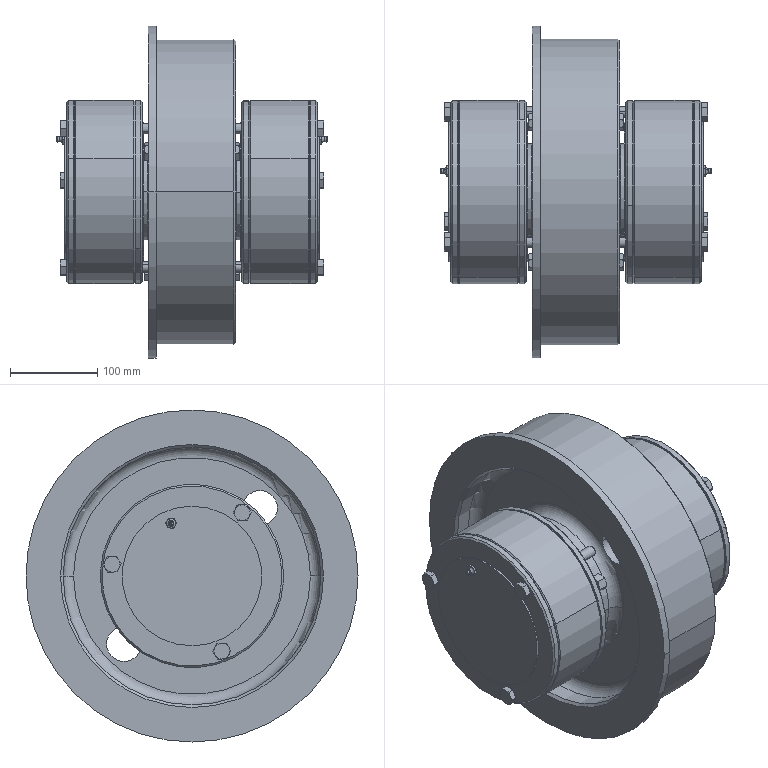Component | SolidWorks | Short-1_L756AngleBoxSingleEdgeWheelSet350-C-3 | 29 solids | 1037 faces | volume 11852495 mm3 | cone 434 | plane 307 | cylinder 234 | torus 62 | commonest cylinder face diameters 13 x36 160 x28 12 x24 110 x20 210 x16 90 x12 114 x12 13.5 x12 | material Plain Carbon Steel